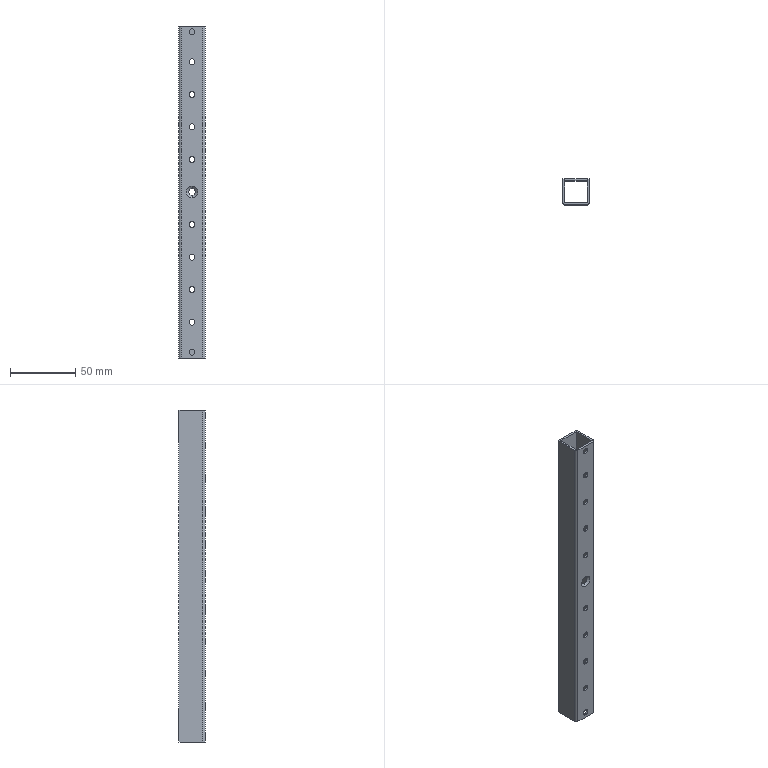Component | SolidWorks | LeftRearDoorAssembly-1_LeftRearDoorWelding-1_RearDoorTransverseStiffener-1 | 3 solids | 56 faces | volume 22487 mm3 | plane 30 | cylinder 24 | cone 2 | commonest cylinder face diameters 4.6 x20 3.2 x2 0.2 x2